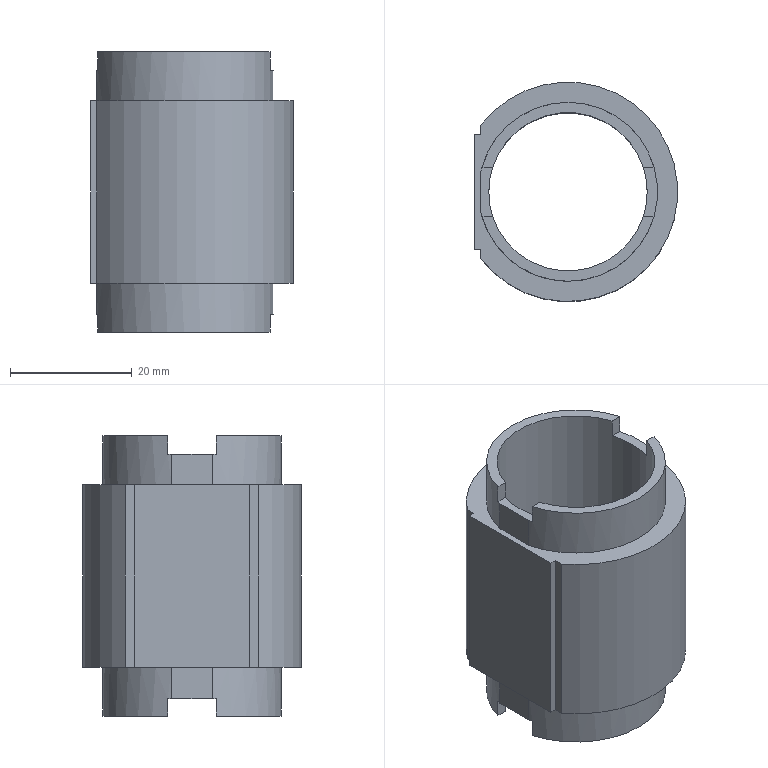Component | NX | 03A__27_2 | 1 solid | 29 faces | volume 15693 mm3 | plane 25 | cylinder 4 | commonest cylinder face diameters 29.376 x2 36 x1 26 x1